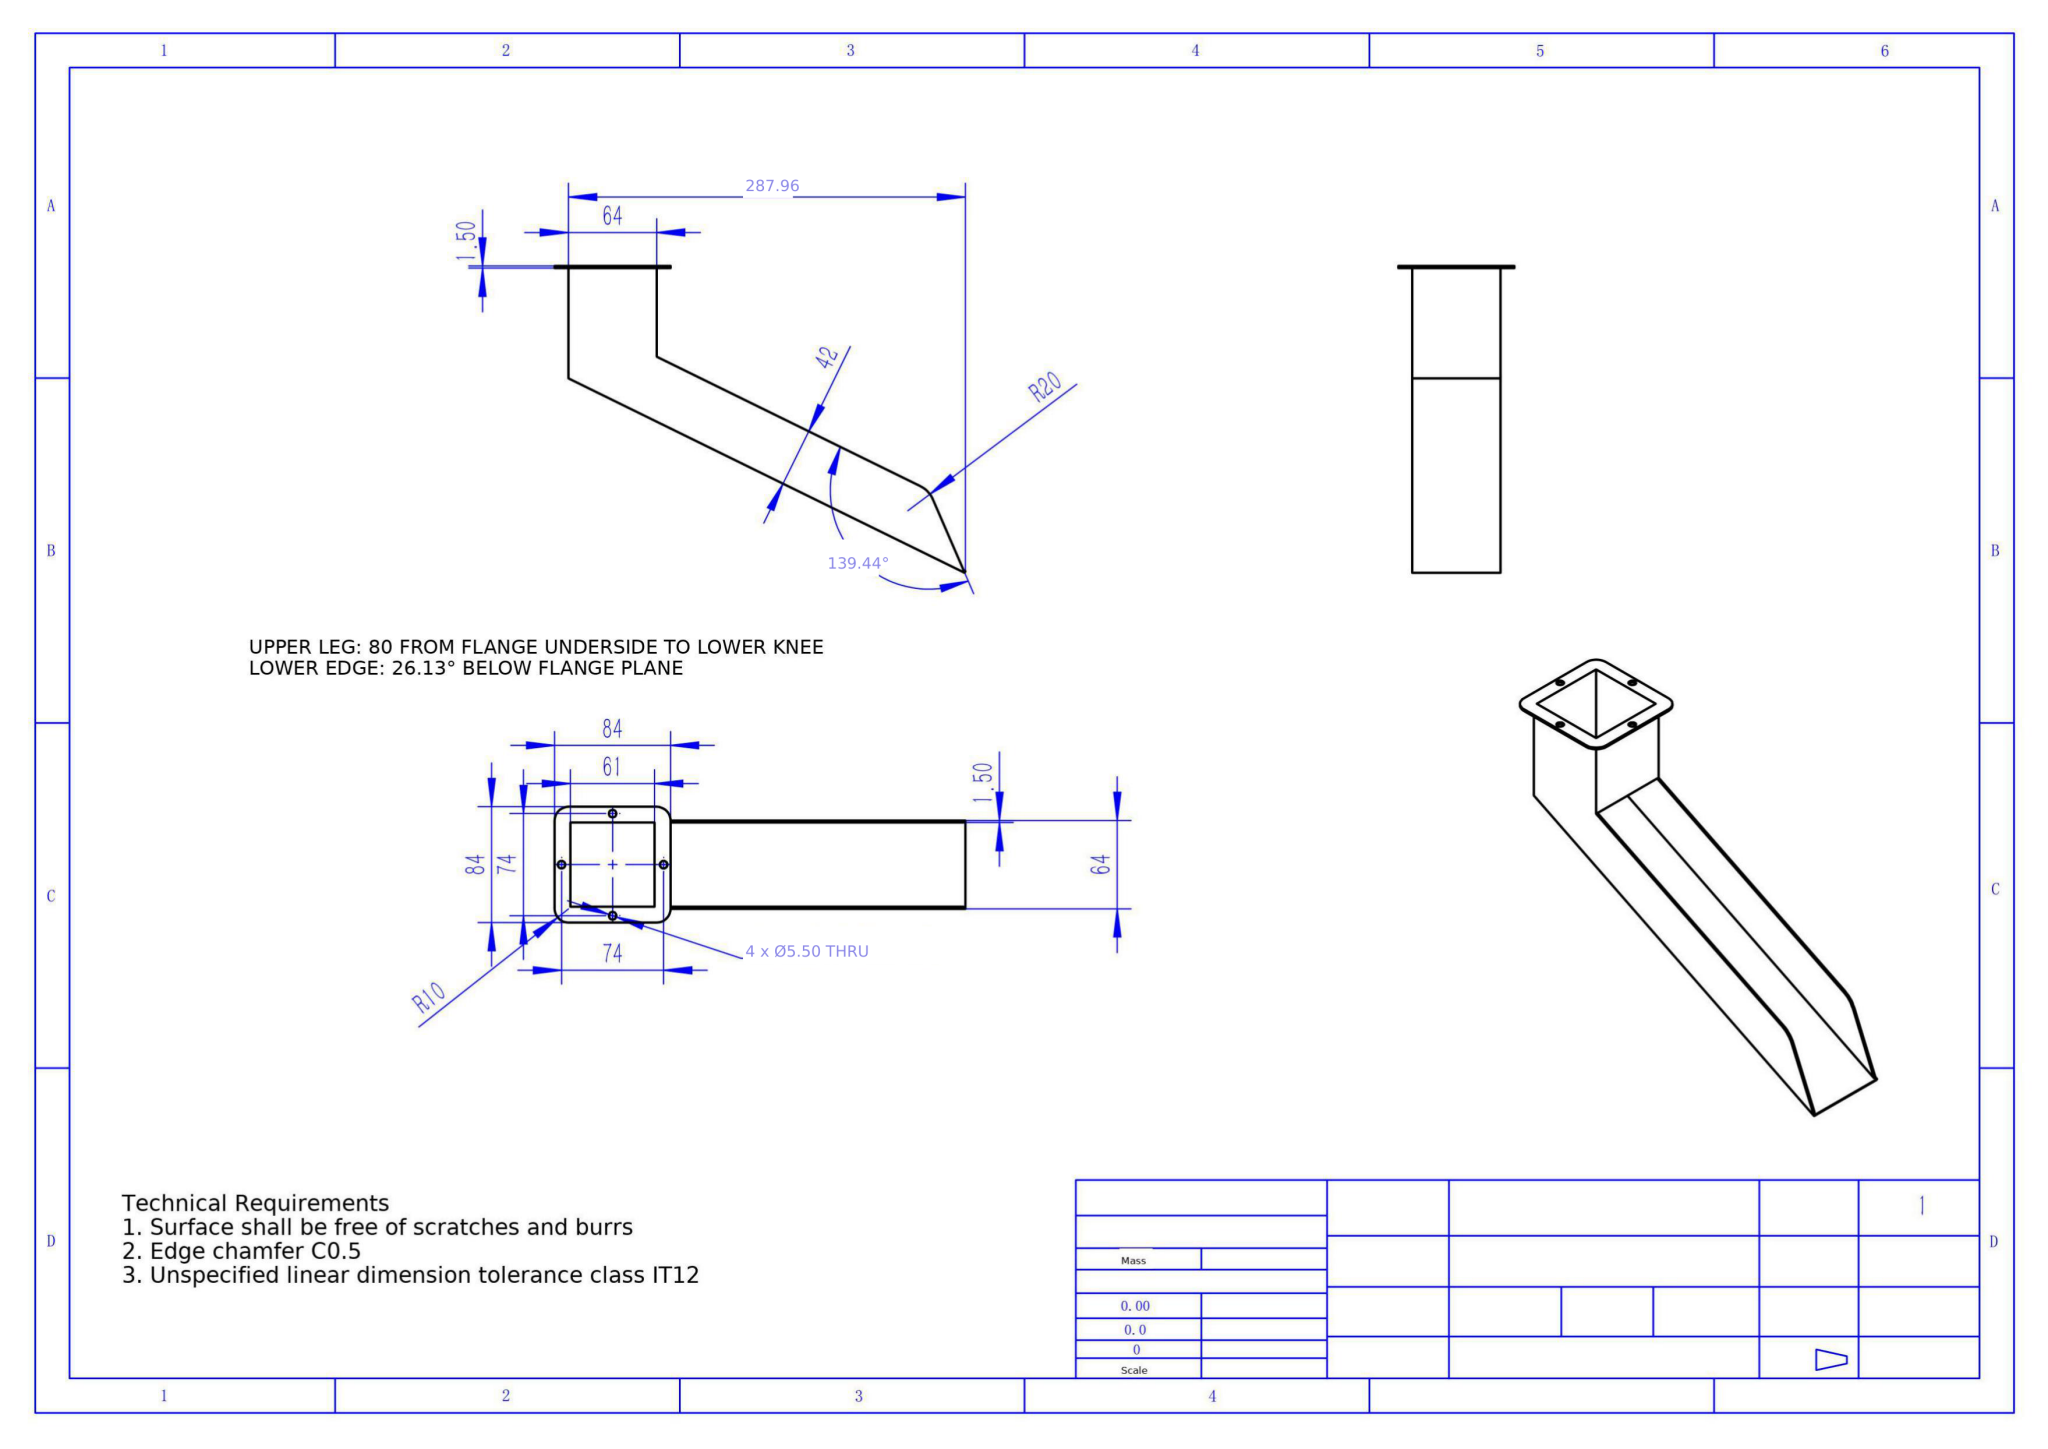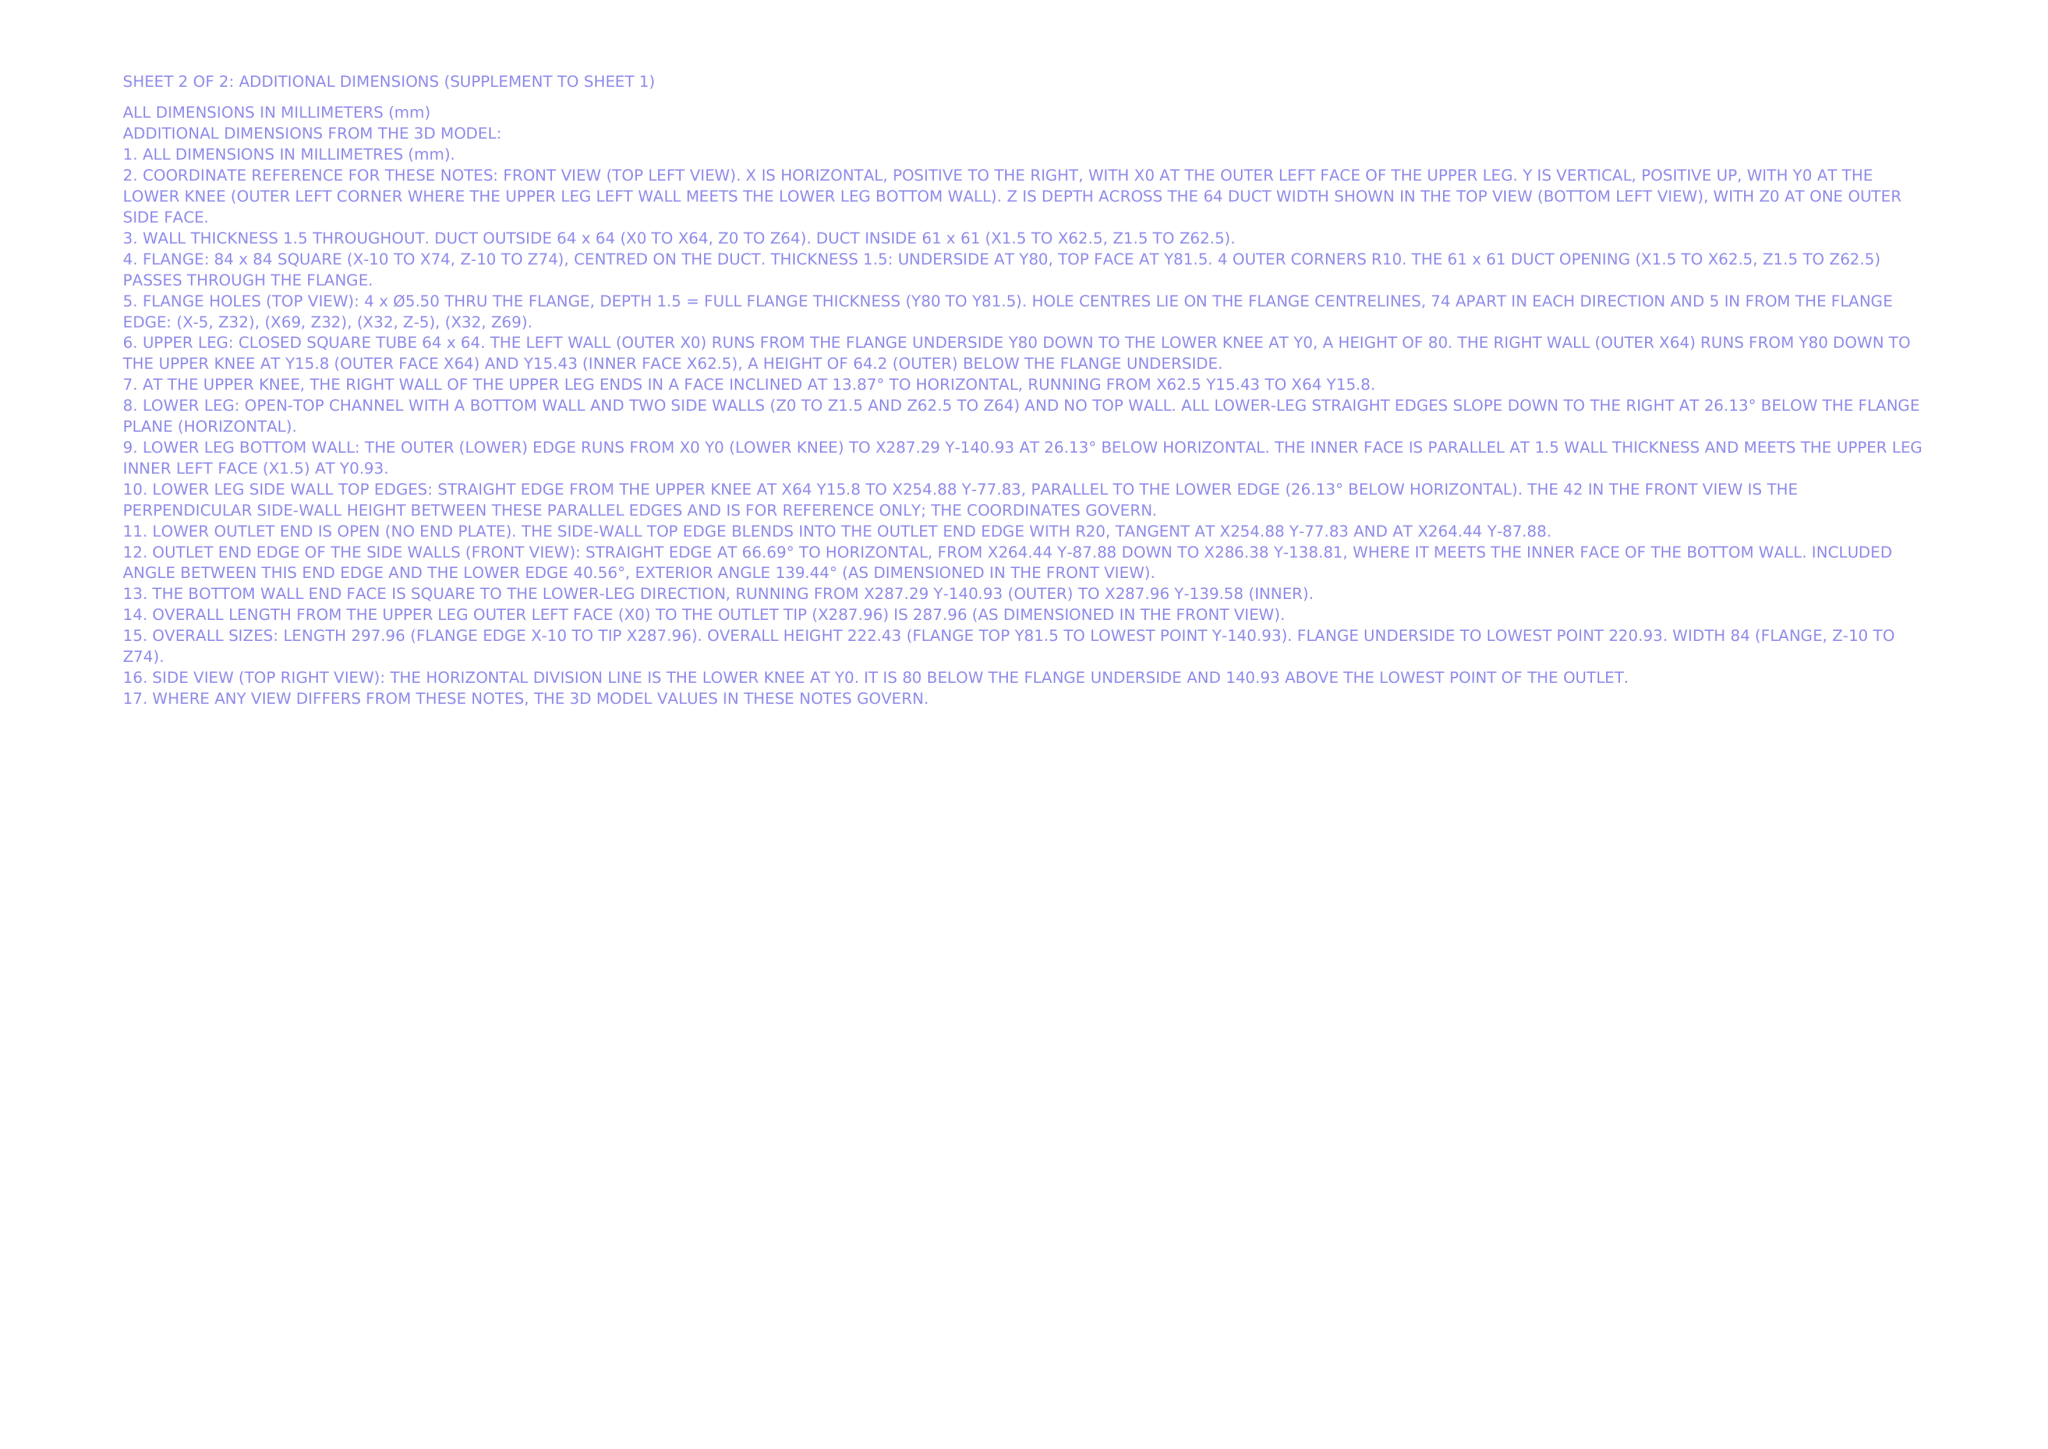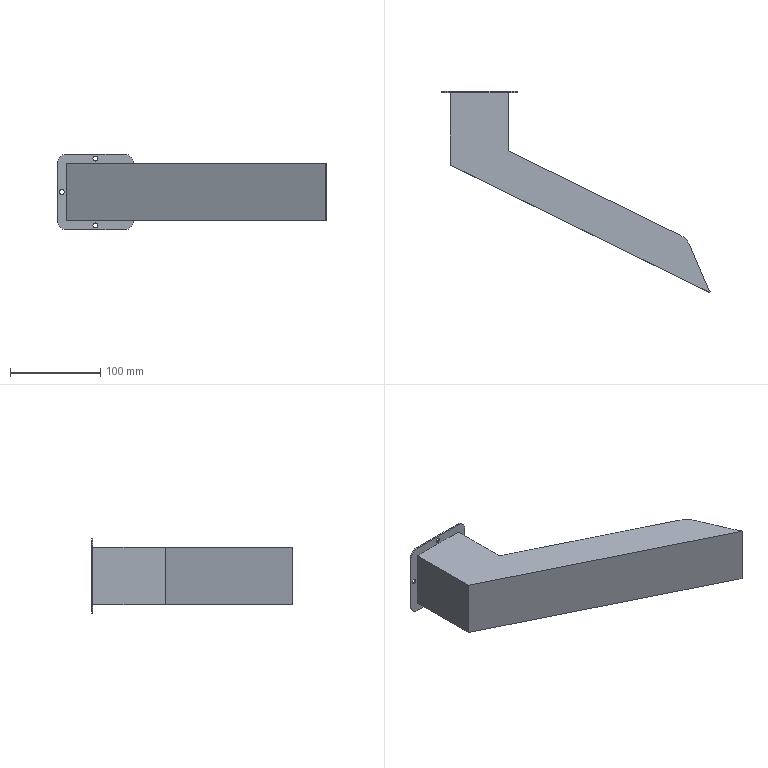Part | NX | mm | Angled Tubular Arm Bracket | 1 solid | 36 faces | box 297.96 x 222.43 x 84 mm | volume 95288 mm3 | plane 22 | cylinder 14 | commonest cylinder face diameters 5.5 x8 20 x4 40 x2